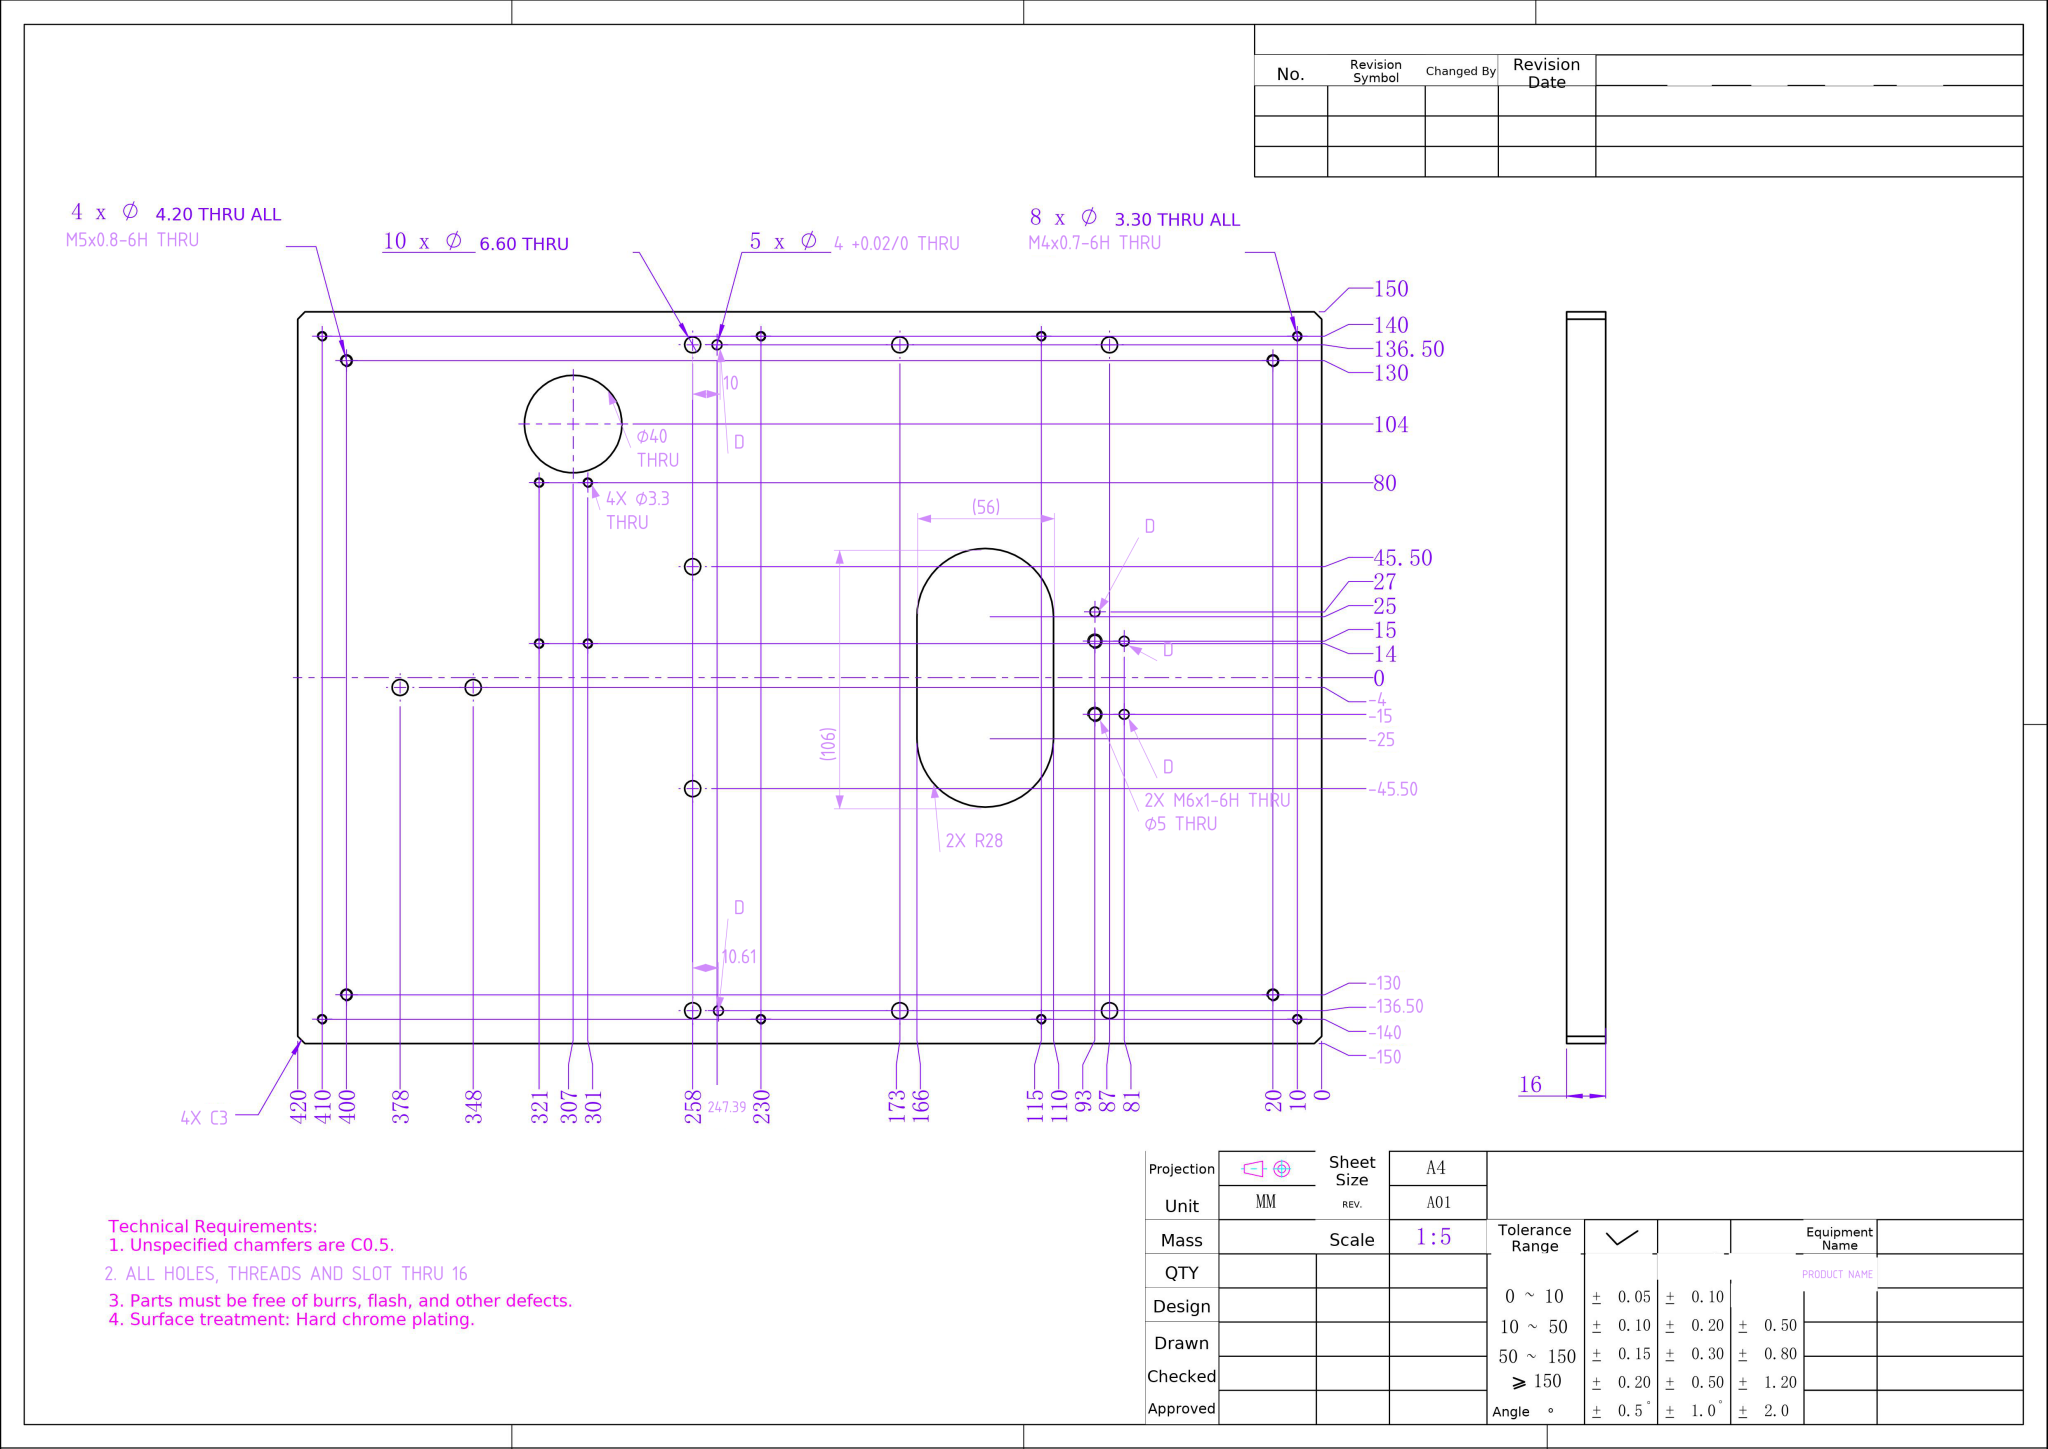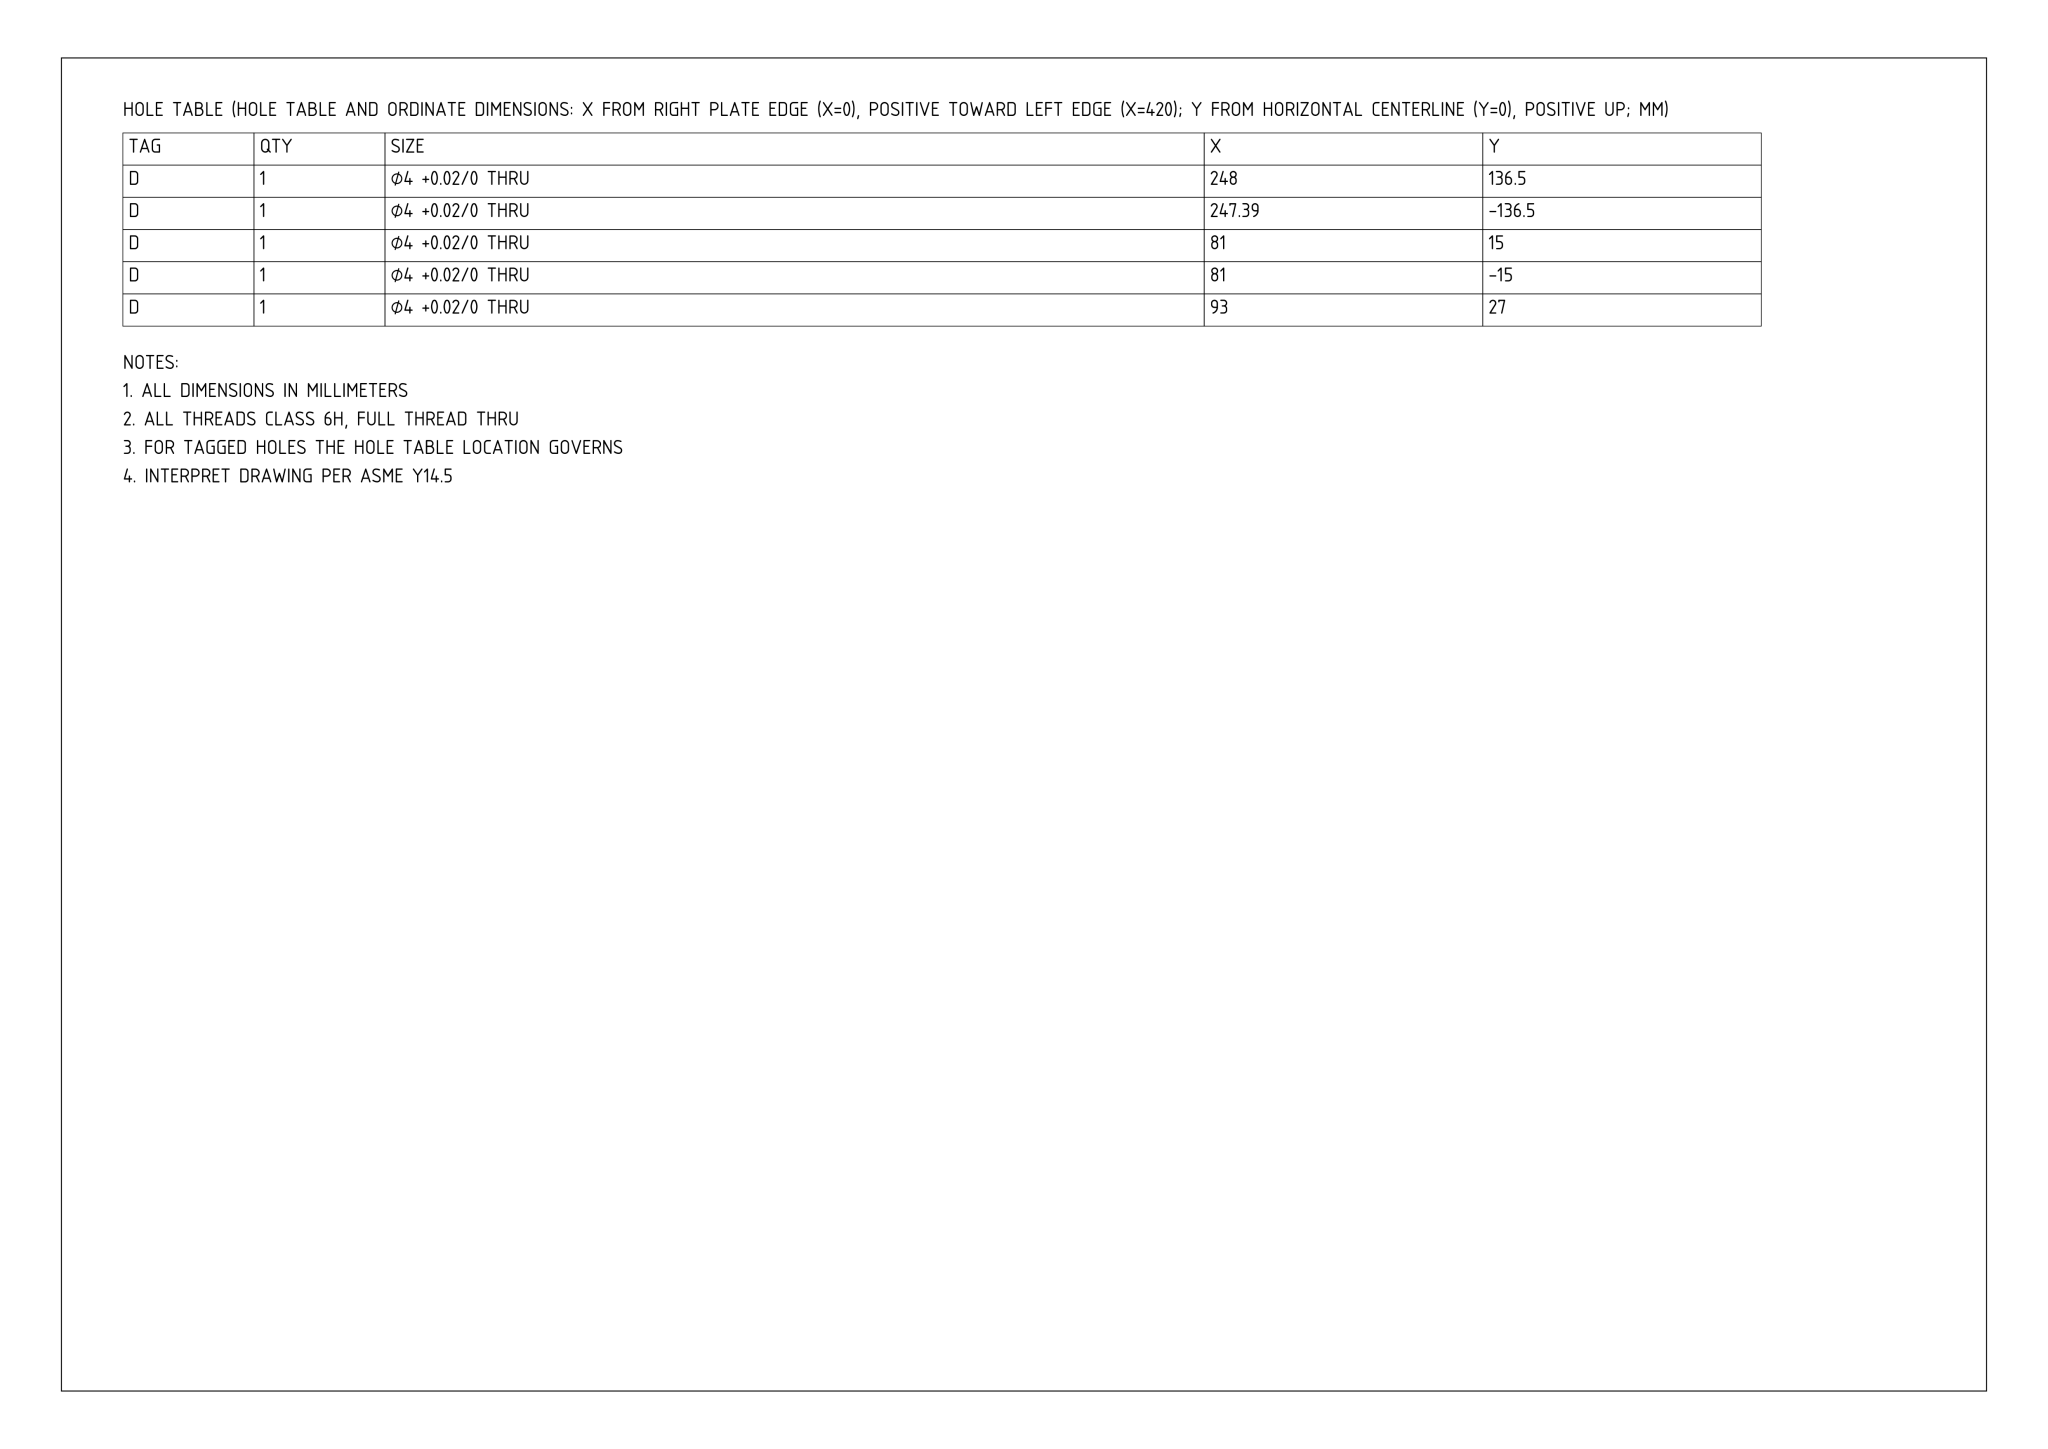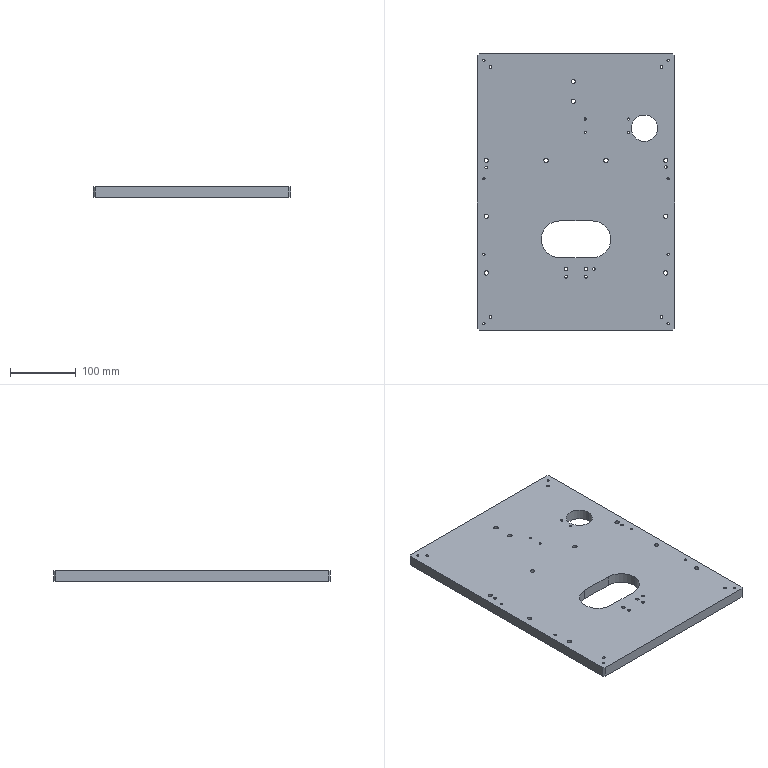Part | NX | mm | 1 solid | 83 faces | box 300 x 420 x 16 mm | volume 1901761 mm3 | cylinder 71 | plane 12 | commonest cylinder face diameters 3.3 x24 6.6 x20 4 x10 4.2 x8 5 x4 56 x3 40 x2